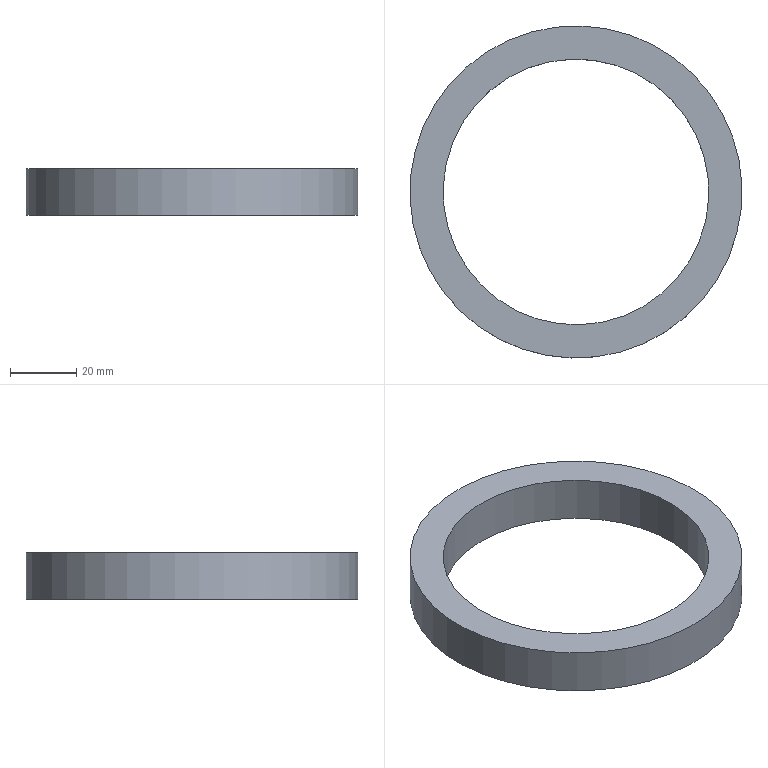Component | NX | CA6140-ZHUZHOU-ZHOUTAO1 | 1 solid | 4 faces | box 100 x 100 x 14 mm | volume 39584 mm3 | plane 2 | cylinder 2 | commonest cylinder face diameters 100 x1 80 x1
STEP:
#1=CARTESIAN_POINT('',(0.,0.,0.));
#2=DIRECTION('',(0.,0.,1.));
#3=DIRECTION('',(1.,0.,0.));
#4=AXIS2_PLACEMENT_3D('',#1,#2,#3);
#5=CARTESIAN_POINT('',(23.511,32.361,-366.451));
#6=VERTEX_POINT('',#5);
#7=CARTESIAN_POINT('',(0.,-0.,-366.451));
#8=DIRECTION('',(0.,0.,-1.));
#9=DIRECTION('',(0.5878,0.809,0.));
#10=AXIS2_PLACEMENT_3D('',#7,#8,#9);
#11=CIRCLE('',#10,40.);
#12=CARTESIAN_POINT('',(0.,-0.,-366.451));
#13=DIRECTION('',(0.,0.,1.));
#14=DIRECTION('',(-0.5878,-0.809,0.));
#15=AXIS2_PLACEMENT_3D('',#12,#13,#14);
#16=PLANE('',#15);
#17=CARTESIAN_POINT('',(-40.,0.));
#18=CARTESIAN_POINT('',(-40.,69.282));
#19=CARTESIAN_POINT('',(20.,34.641));
#20=CARTESIAN_POINT('',(80.,0.));
#21=CARTESIAN_POINT('',(20.,-34.641));
#22=CARTESIAN_POINT('',(-40.,-69.282));
#23=CARTESIAN_POINT('',(-40.,0.));
#24=(BOUNDED_CURVE()B_SPLINE_CURVE(2,(#17,#18,#19,#20,#21,#22,#23),.UNSPECIFIED.,.T.,.F.)B_SPLINE_CURVE_WITH_KNOTS((1,2,2,2,2,1),(-2.094,0.,2.094,4.189,6.283,8.378),.UNSPECIFIED.)CURVE()GEOMETRIC_REPRESENTATION_ITEM()RATIONAL_B_SPLINE_CURVE((1.,0.5,1.,0.5,1.,0.5,1.))REPRESENTATION_ITEM(''));
#25=(GEOMETRIC_REPRESENTATION_CONTEXT(2)PARAMETRIC_REPRESENTATION_CONTEXT()REPRESENTATION_CONTEXT('',''));
#26=DEFINITIONAL_REPRESENTATION('',(#24),#25);
#27=PCURVE('',#16,#26);
#28=CARTESIAN_POINT('',(0.,-0.,-366.451));
#29=DIRECTION('',(0.,0.,-1.));
#30=DIRECTION('',(0.5878,0.809,0.));
#31=AXIS2_PLACEMENT_3D('',#28,#29,#30);
#32=CYLINDRICAL_SURFACE('',#31,40.);
#33=CARTESIAN_POINT('',(0.,0.));
#34=DIRECTION('',(1.,0.));
#35=VECTOR('',#34,1.);
#36=LINE('',#33,#35);
#37=(GEOMETRIC_REPRESENTATION_CONTEXT(2)PARAMETRIC_REPRESENTATION_CONTEXT()REPRESENTATION_CONTEXT('',''));
#38=DEFINITIONAL_REPRESENTATION('',(#36),#37);
#39=PCURVE('',#32,#38);
#40=SURFACE_CURVE('',#11,(#27,#39),.PCURVE_S1.);
#41=EDGE_CURVE('',#6,#6,#40,.T.);
#42=ORIENTED_EDGE('',*,*,#41,.T.);
#43=EDGE_LOOP('',(#42));
#44=FACE_BOUND('',#43,.T.);
#45=CARTESIAN_POINT('',(29.389,40.451,-366.451));
#46=VERTEX_POINT('',#45);
#47=CARTESIAN_POINT('',(-29.389,-40.451,-366.451));
#48=VERTEX_POINT('',#47);
#49=CARTESIAN_POINT('',(0.,-0.,-366.451));
#50=DIRECTION('',(0.,0.,-1.));
#51=DIRECTION('',(0.5878,0.809,0.));
#52=AXIS2_PLACEMENT_3D('',#49,#50,#51);
#53=CIRCLE('',#52,50.);
#54=CARTESIAN_POINT('',(-50.,0.));
#55=CARTESIAN_POINT('',(-50.,86.603));
#56=CARTESIAN_POINT('',(25.,43.301));
#57=CARTESIAN_POINT('',(100.,0.));
#58=CARTESIAN_POINT('',(25.,-43.301));
#59=CARTESIAN_POINT('',(-50.,-86.603));
#60=CARTESIAN_POINT('',(-50.,0.));
#61=(BOUNDED_CURVE()B_SPLINE_CURVE(2,(#54,#55,#56,#57,#58,#59,#60),.UNSPECIFIED.,.T.,.F.)B_SPLINE_CURVE_WITH_KNOTS((1,2,2,2,2,1),(-2.094,0.,2.094,4.189,6.283,8.378),.UNSPECIFIED.)CURVE()GEOMETRIC_REPRESENTATION_ITEM()RATIONAL_B_SPLINE_CURVE((1.,0.5,1.,0.5,1.,0.5,1.))REPRESENTATION_ITEM(''));
#62=(GEOMETRIC_REPRESENTATION_CONTEXT(2)PARAMETRIC_REPRESENTATION_CONTEXT()REPRESENTATION_CONTEXT('',''));
#63=DEFINITIONAL_REPRESENTATION('',(#61),#62);
#64=PCURVE('',#16,#63);
#65=CARTESIAN_POINT('',(0.,-0.,-380.451));
#66=DIRECTION('',(0.,0.,1.));
#67=DIRECTION('',(-0.5878,-0.809,0.));
#68=AXIS2_PLACEMENT_3D('',#65,#66,#67);
#69=CYLINDRICAL_SURFACE('',#68,50.);
#70=CARTESIAN_POINT('',(3.142,14.));
#71=DIRECTION('',(-1.,0.));
#72=VECTOR('',#71,1.);
#73=LINE('',#70,#72);
#74=(GEOMETRIC_REPRESENTATION_CONTEXT(2)PARAMETRIC_REPRESENTATION_CONTEXT()REPRESENTATION_CONTEXT('',''));
#75=DEFINITIONAL_REPRESENTATION('',(#73),#74);
#76=PCURVE('',#69,#75);
#77=SURFACE_CURVE('',#53,(#64,#76),.PCURVE_S1.);
#78=EDGE_CURVE('',#46,#48,#77,.T.);
#79=ORIENTED_EDGE('',*,*,#78,.F.);
#80=CARTESIAN_POINT('',(0.,-0.,-366.451));
#81=DIRECTION('',(0.,0.,-1.));
#82=DIRECTION('',(0.5878,0.809,0.));
#83=AXIS2_PLACEMENT_3D('',#80,#81,#82);
#84=CIRCLE('',#83,50.);
#85=CARTESIAN_POINT('',(-50.,0.));
#86=CARTESIAN_POINT('',(-50.,86.603));
#87=CARTESIAN_POINT('',(25.,43.301));
#88=CARTESIAN_POINT('',(100.,0.));
#89=CARTESIAN_POINT('',(25.,-43.301));
#90=CARTESIAN_POINT('',(-50.,-86.603));
#91=CARTESIAN_POINT('',(-50.,0.));
#92=(BOUNDED_CURVE()B_SPLINE_CURVE(2,(#85,#86,#87,#88,#89,#90,#91),.UNSPECIFIED.,.T.,.F.)B_SPLINE_CURVE_WITH_KNOTS((1,2,2,2,2,1),(-2.094,0.,2.094,4.189,6.283,8.378),.UNSPECIFIED.)CURVE()GEOMETRIC_REPRESENTATION_ITEM()RATIONAL_B_SPLINE_CURVE((1.,0.5,1.,0.5,1.,0.5,1.))REPRESENTATION_ITEM(''));
#93=(GEOMETRIC_REPRESENTATION_CONTEXT(2)PARAMETRIC_REPRESENTATION_CONTEXT()REPRESENTATION_CONTEXT('',''));
#94=DEFINITIONAL_REPRESENTATION('',(#92),#93);
#95=PCURVE('',#16,#94);
#96=CARTESIAN_POINT('',(9.425,14.));
#97=DIRECTION('',(-1.,0.));
#98=VECTOR('',#97,1.);
#99=LINE('',#96,#98);
#100=(GEOMETRIC_REPRESENTATION_CONTEXT(2)PARAMETRIC_REPRESENTATION_CONTEXT()REPRESENTATION_CONTEXT('',''));
#101=DEFINITIONAL_REPRESENTATION('',(#99),#100);
#102=PCURVE('',#69,#101);
#103=SURFACE_CURVE('',#84,(#95,#102),.PCURVE_S1.);
#104=EDGE_CURVE('',#48,#46,#103,.T.);
#105=ORIENTED_EDGE('',*,*,#104,.F.);
#106=EDGE_LOOP('',(#79,#105));
#107=FACE_BOUND('',#106,.T.);
#108=ADVANCED_FACE('',(#44,#107),#16,.T.);
#109=CARTESIAN_POINT('',(23.511,32.361,-380.451));
#110=VERTEX_POINT('',#109);
#111=CARTESIAN_POINT('',(0.,-0.,-380.451));
#112=DIRECTION('',(0.,0.,-1.));
#113=DIRECTION('',(0.5878,0.809,0.));
#114=AXIS2_PLACEMENT_3D('',#111,#112,#113);
#115=CIRCLE('',#114,40.);
#116=CARTESIAN_POINT('',(0.,-0.,-380.451));
#117=DIRECTION('',(0.,0.,-1.));
#118=DIRECTION('',(0.5878,0.809,0.));
#119=AXIS2_PLACEMENT_3D('',#116,#117,#118);
#120=PLANE('',#119);
#121=CARTESIAN_POINT('',(0.,0.));
#122=DIRECTION('',(1.,0.));
#123=AXIS2_PLACEMENT_2D('',#121,#122);
#124=CIRCLE('',#123,40.);
#125=(GEOMETRIC_REPRESENTATION_CONTEXT(2)PARAMETRIC_REPRESENTATION_CONTEXT()REPRESENTATION_CONTEXT('',''));
#126=DEFINITIONAL_REPRESENTATION('',(#124),#125);
#127=PCURVE('',#120,#126);
#128=CARTESIAN_POINT('',(0.,14.));
#129=DIRECTION('',(1.,0.));
#130=VECTOR('',#129,1.);
#131=LINE('',#128,#130);
#132=(GEOMETRIC_REPRESENTATION_CONTEXT(2)PARAMETRIC_REPRESENTATION_CONTEXT()REPRESENTATION_CONTEXT('',''));
#133=DEFINITIONAL_REPRESENTATION('',(#131),#132);
#134=PCURVE('',#32,#133);
#135=SURFACE_CURVE('',#115,(#127,#134),.PCURVE_S1.);
#136=EDGE_CURVE('',#110,#110,#135,.T.);
#137=ORIENTED_EDGE('',*,*,#136,.F.);
#138=EDGE_LOOP('',(#137));
#139=FACE_BOUND('',#138,.T.);
#140=CARTESIAN_POINT('',(-29.389,-40.451,-380.451));
#141=VERTEX_POINT('',#140);
#142=CARTESIAN_POINT('',(0.,-0.,-380.451));
#143=DIRECTION('',(0.,0.,1.));
#144=DIRECTION('',(-0.5878,-0.809,0.));
#145=AXIS2_PLACEMENT_3D('',#142,#143,#144);
#146=CIRCLE('',#145,50.);
#147=CARTESIAN_POINT('',(-50.,0.));
#148=CARTESIAN_POINT('',(-50.,86.603));
#149=CARTESIAN_POINT('',(25.,43.301));
#150=CARTESIAN_POINT('',(100.,0.));
#151=CARTESIAN_POINT('',(25.,-43.301));
#152=CARTESIAN_POINT('',(-50.,-86.603));
#153=CARTESIAN_POINT('',(-50.,0.));
#154=(BOUNDED_CURVE()B_SPLINE_CURVE(2,(#147,#148,#149,#150,#151,#152,#153),.UNSPECIFIED.,.T.,.F.)B_SPLINE_CURVE_WITH_KNOTS((1,2,2,2,2,1),(-2.094,0.,2.094,4.189,6.283,8.378),.UNSPECIFIED.)CURVE()GEOMETRIC_REPRESENTATION_ITEM()RATIONAL_B_SPLINE_CURVE((1.,0.5,1.,0.5,1.,0.5,1.))REPRESENTATION_ITEM(''));
#155=(GEOMETRIC_REPRESENTATION_CONTEXT(2)PARAMETRIC_REPRESENTATION_CONTEXT()REPRESENTATION_CONTEXT('',''));
#156=DEFINITIONAL_REPRESENTATION('',(#154),#155);
#157=PCURVE('',#120,#156);
#158=CARTESIAN_POINT('',(0.,0.));
#159=DIRECTION('',(1.,0.));
#160=VECTOR('',#159,1.);
#161=LINE('',#158,#160);
#162=(GEOMETRIC_REPRESENTATION_CONTEXT(2)PARAMETRIC_REPRESENTATION_CONTEXT()REPRESENTATION_CONTEXT('',''));
#163=DEFINITIONAL_REPRESENTATION('',(#161),#162);
#164=PCURVE('',#69,#163);
#165=SURFACE_CURVE('',#146,(#157,#164),.PCURVE_S1.);
#166=EDGE_CURVE('',#141,#141,#165,.T.);
#167=ORIENTED_EDGE('',*,*,#166,.F.);
#168=EDGE_LOOP('',(#167));
#169=FACE_BOUND('',#168,.T.);
#170=ADVANCED_FACE('',(#139,#169),#120,.T.);
#171=ORIENTED_EDGE('',*,*,#78,.T.);
#172=CARTESIAN_POINT('',(-29.389,-40.451,-380.451));
#173=CARTESIAN_POINT('',(-29.389,-40.451,-366.451));
#174=B_SPLINE_CURVE_WITH_KNOTS('',1,(#172,#173),.UNSPECIFIED.,.F.,.F.,(2,2),(0.,14.),.PIECEWISE_BEZIER_KNOTS.);
#175=CARTESIAN_POINT('',(0.,0.));
#176=DIRECTION('',(0.,1.));
#177=VECTOR('',#176,1.);
#178=LINE('',#175,#177);
#179=(GEOMETRIC_REPRESENTATION_CONTEXT(2)PARAMETRIC_REPRESENTATION_CONTEXT()REPRESENTATION_CONTEXT('',''));
#180=DEFINITIONAL_REPRESENTATION('',(#178),#179);
#181=PCURVE('',#69,#180);
#182=CARTESIAN_POINT('',(6.283,0.));
#183=DIRECTION('',(0.,1.));
#184=VECTOR('',#183,1.);
#185=LINE('',#182,#184);
#186=(GEOMETRIC_REPRESENTATION_CONTEXT(2)PARAMETRIC_REPRESENTATION_CONTEXT()REPRESENTATION_CONTEXT('',''));
#187=DEFINITIONAL_REPRESENTATION('',(#185),#186);
#188=PCURVE('',#69,#187);
#189=SEAM_CURVE('',#174,(#181,#188),.PCURVE_S1.);
#190=EDGE_CURVE('',#141,#48,#189,.T.);
#191=ORIENTED_EDGE('',*,*,#190,.F.);
#192=ORIENTED_EDGE('',*,*,#166,.T.);
#193=ORIENTED_EDGE('',*,*,#190,.T.);
#194=ORIENTED_EDGE('',*,*,#104,.T.);
#195=EDGE_LOOP('',(#171,#191,#192,#193,#194));
#196=FACE_BOUND('',#195,.T.);
#197=ADVANCED_FACE('',(#196),#69,.T.);
#198=ORIENTED_EDGE('',*,*,#136,.F.);
#199=CARTESIAN_POINT('',(23.511,32.361,-366.451));
#200=CARTESIAN_POINT('',(23.511,32.361,-380.451));
#201=B_SPLINE_CURVE_WITH_KNOTS('',1,(#199,#200),.UNSPECIFIED.,.F.,.F.,(2,2),(0.,14.),.PIECEWISE_BEZIER_KNOTS.);
#202=CARTESIAN_POINT('',(0.,0.));
#203=DIRECTION('',(0.,1.));
#204=VECTOR('',#203,1.);
#205=LINE('',#202,#204);
#206=(GEOMETRIC_REPRESENTATION_CONTEXT(2)PARAMETRIC_REPRESENTATION_CONTEXT()REPRESENTATION_CONTEXT('',''));
#207=DEFINITIONAL_REPRESENTATION('',(#205),#206);
#208=PCURVE('',#32,#207);
#209=CARTESIAN_POINT('',(6.283,0.));
#210=DIRECTION('',(0.,1.));
#211=VECTOR('',#210,1.);
#212=LINE('',#209,#211);
#213=(GEOMETRIC_REPRESENTATION_CONTEXT(2)PARAMETRIC_REPRESENTATION_CONTEXT()REPRESENTATION_CONTEXT('',''));
#214=DEFINITIONAL_REPRESENTATION('',(#212),#213);
#215=PCURVE('',#32,#214);
#216=SEAM_CURVE('',#201,(#208,#215),.PCURVE_S1.);
#217=EDGE_CURVE('',#6,#110,#216,.T.);
#218=ORIENTED_EDGE('',*,*,#217,.F.);
#219=ORIENTED_EDGE('',*,*,#41,.T.);
#220=ORIENTED_EDGE('',*,*,#217,.T.);
#221=EDGE_LOOP('',(#198,#218,#219,#220));
#222=FACE_BOUND('',#221,.F.);
#223=ADVANCED_FACE('',(#222),#32,.F.);
#224=CLOSED_SHELL('',(#108,#170,#197,#223));
#225=MANIFOLD_SOLID_BREP('',#224);
#226=(LENGTH_UNIT()NAMED_UNIT(*)SI_UNIT(.MILLI.,.METRE.));
#227=UNCERTAINTY_MEASURE_WITH_UNIT(LENGTH_MEASURE(0.000005),#226,'','');
#228=(NAMED_UNIT(*)PLANE_ANGLE_UNIT()SI_UNIT($,.RADIAN.));
#229=(NAMED_UNIT(*)SI_UNIT($,.STERADIAN.)SOLID_ANGLE_UNIT());
#230=(GEOMETRIC_REPRESENTATION_CONTEXT(3)GLOBAL_UNCERTAINTY_ASSIGNED_CONTEXT((#227))GLOBAL_UNIT_ASSIGNED_CONTEXT((#226,#228,#229))REPRESENTATION_CONTEXT('',''));
#231=ADVANCED_BREP_SHAPE_REPRESENTATION('',(#4,#225),#230);